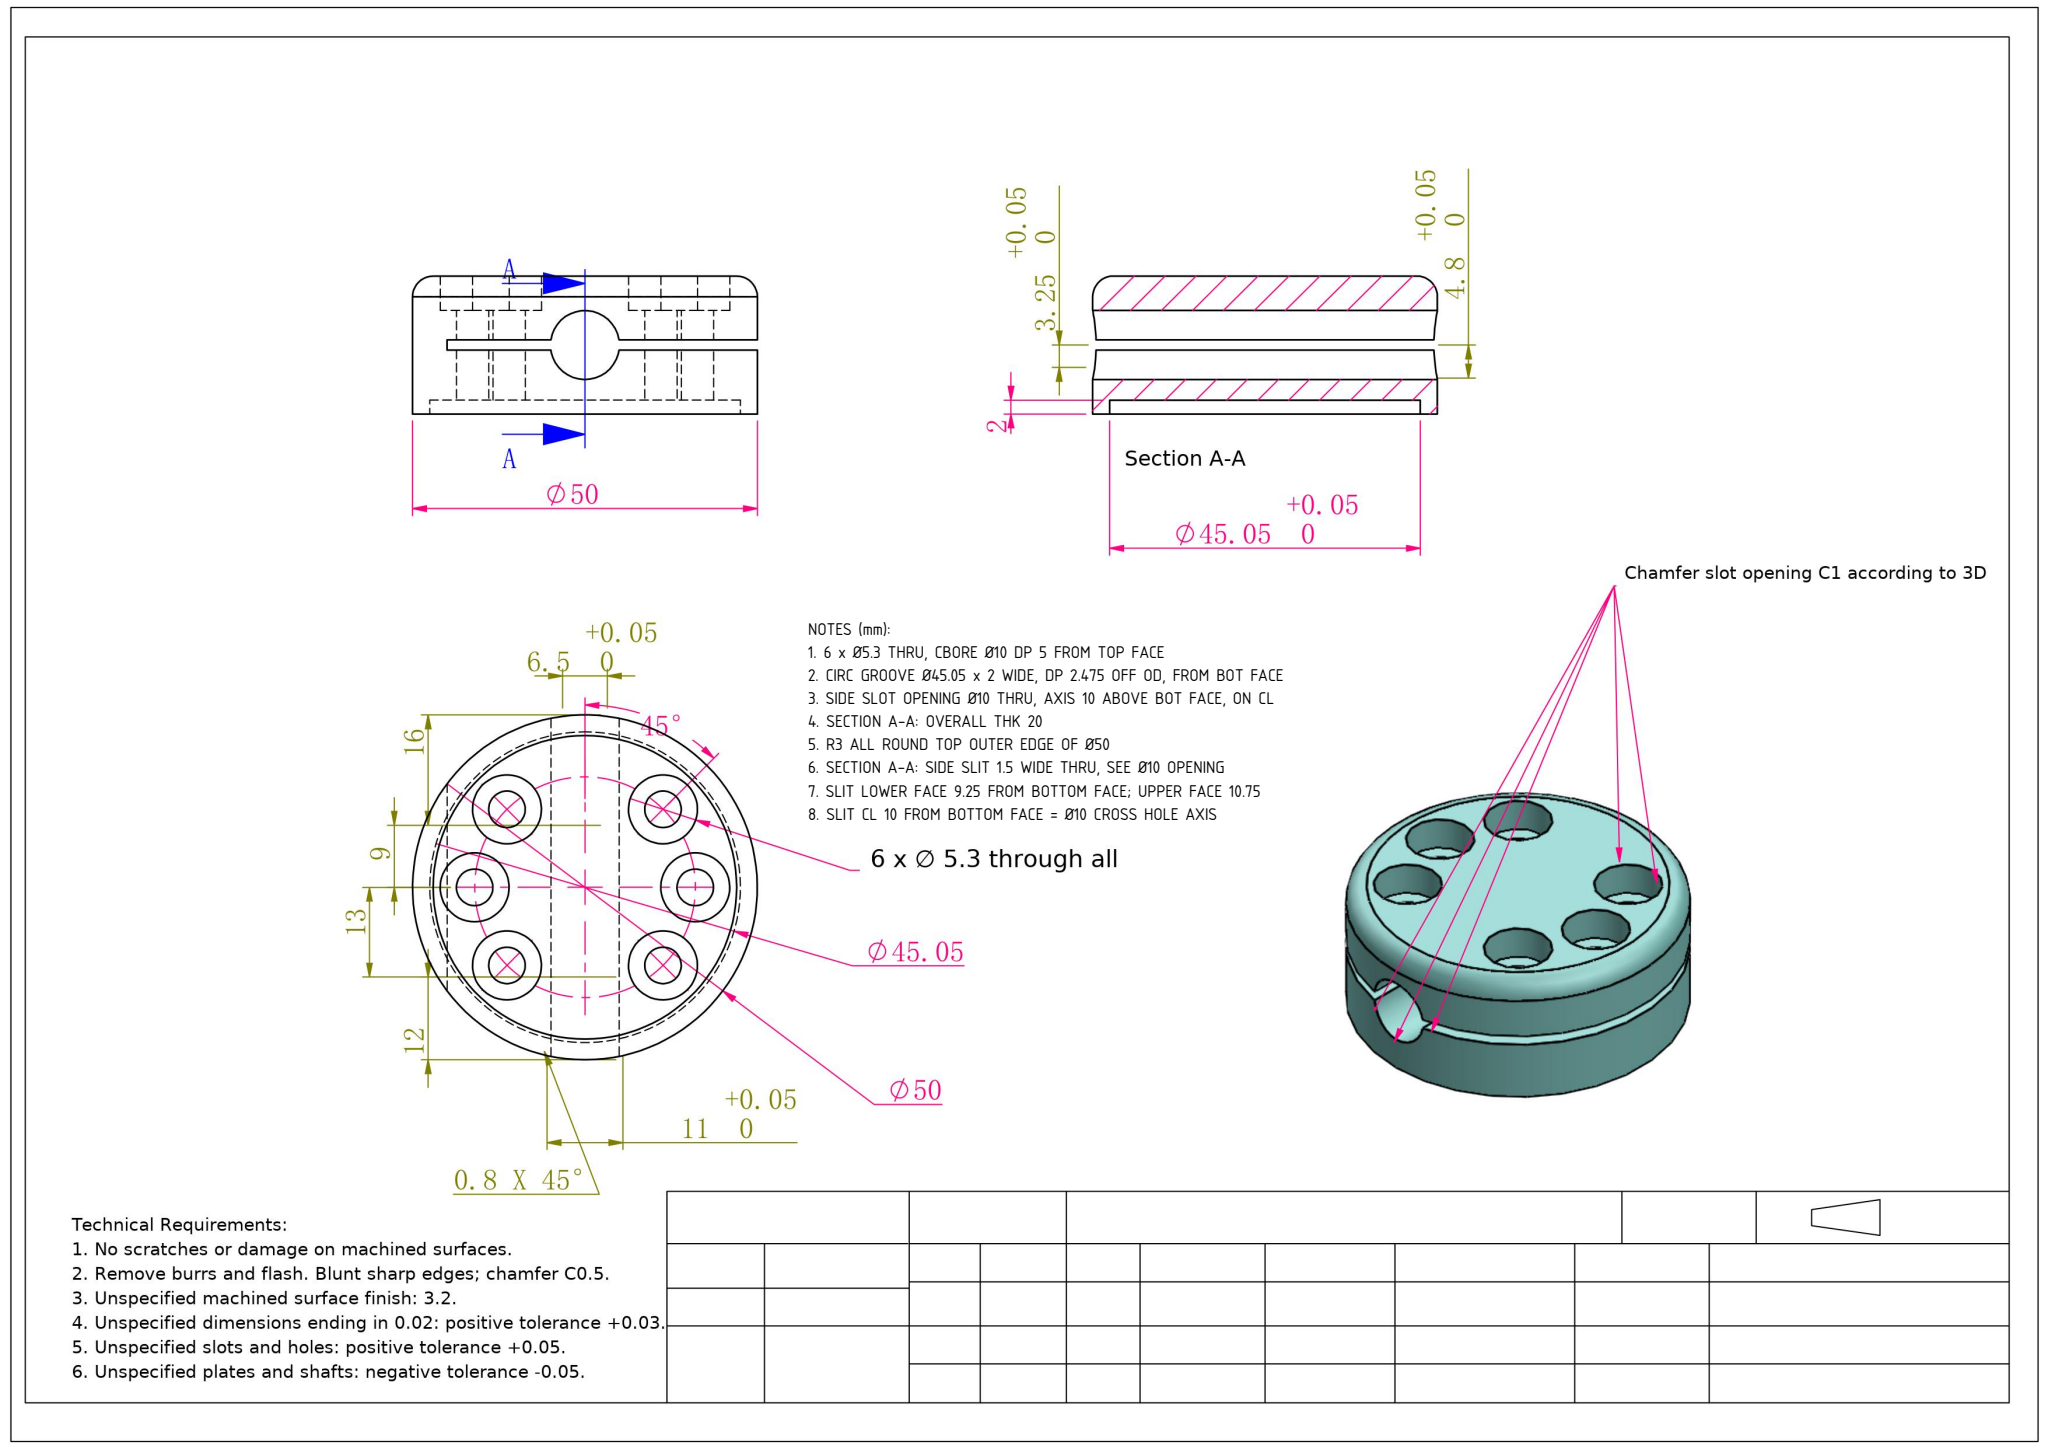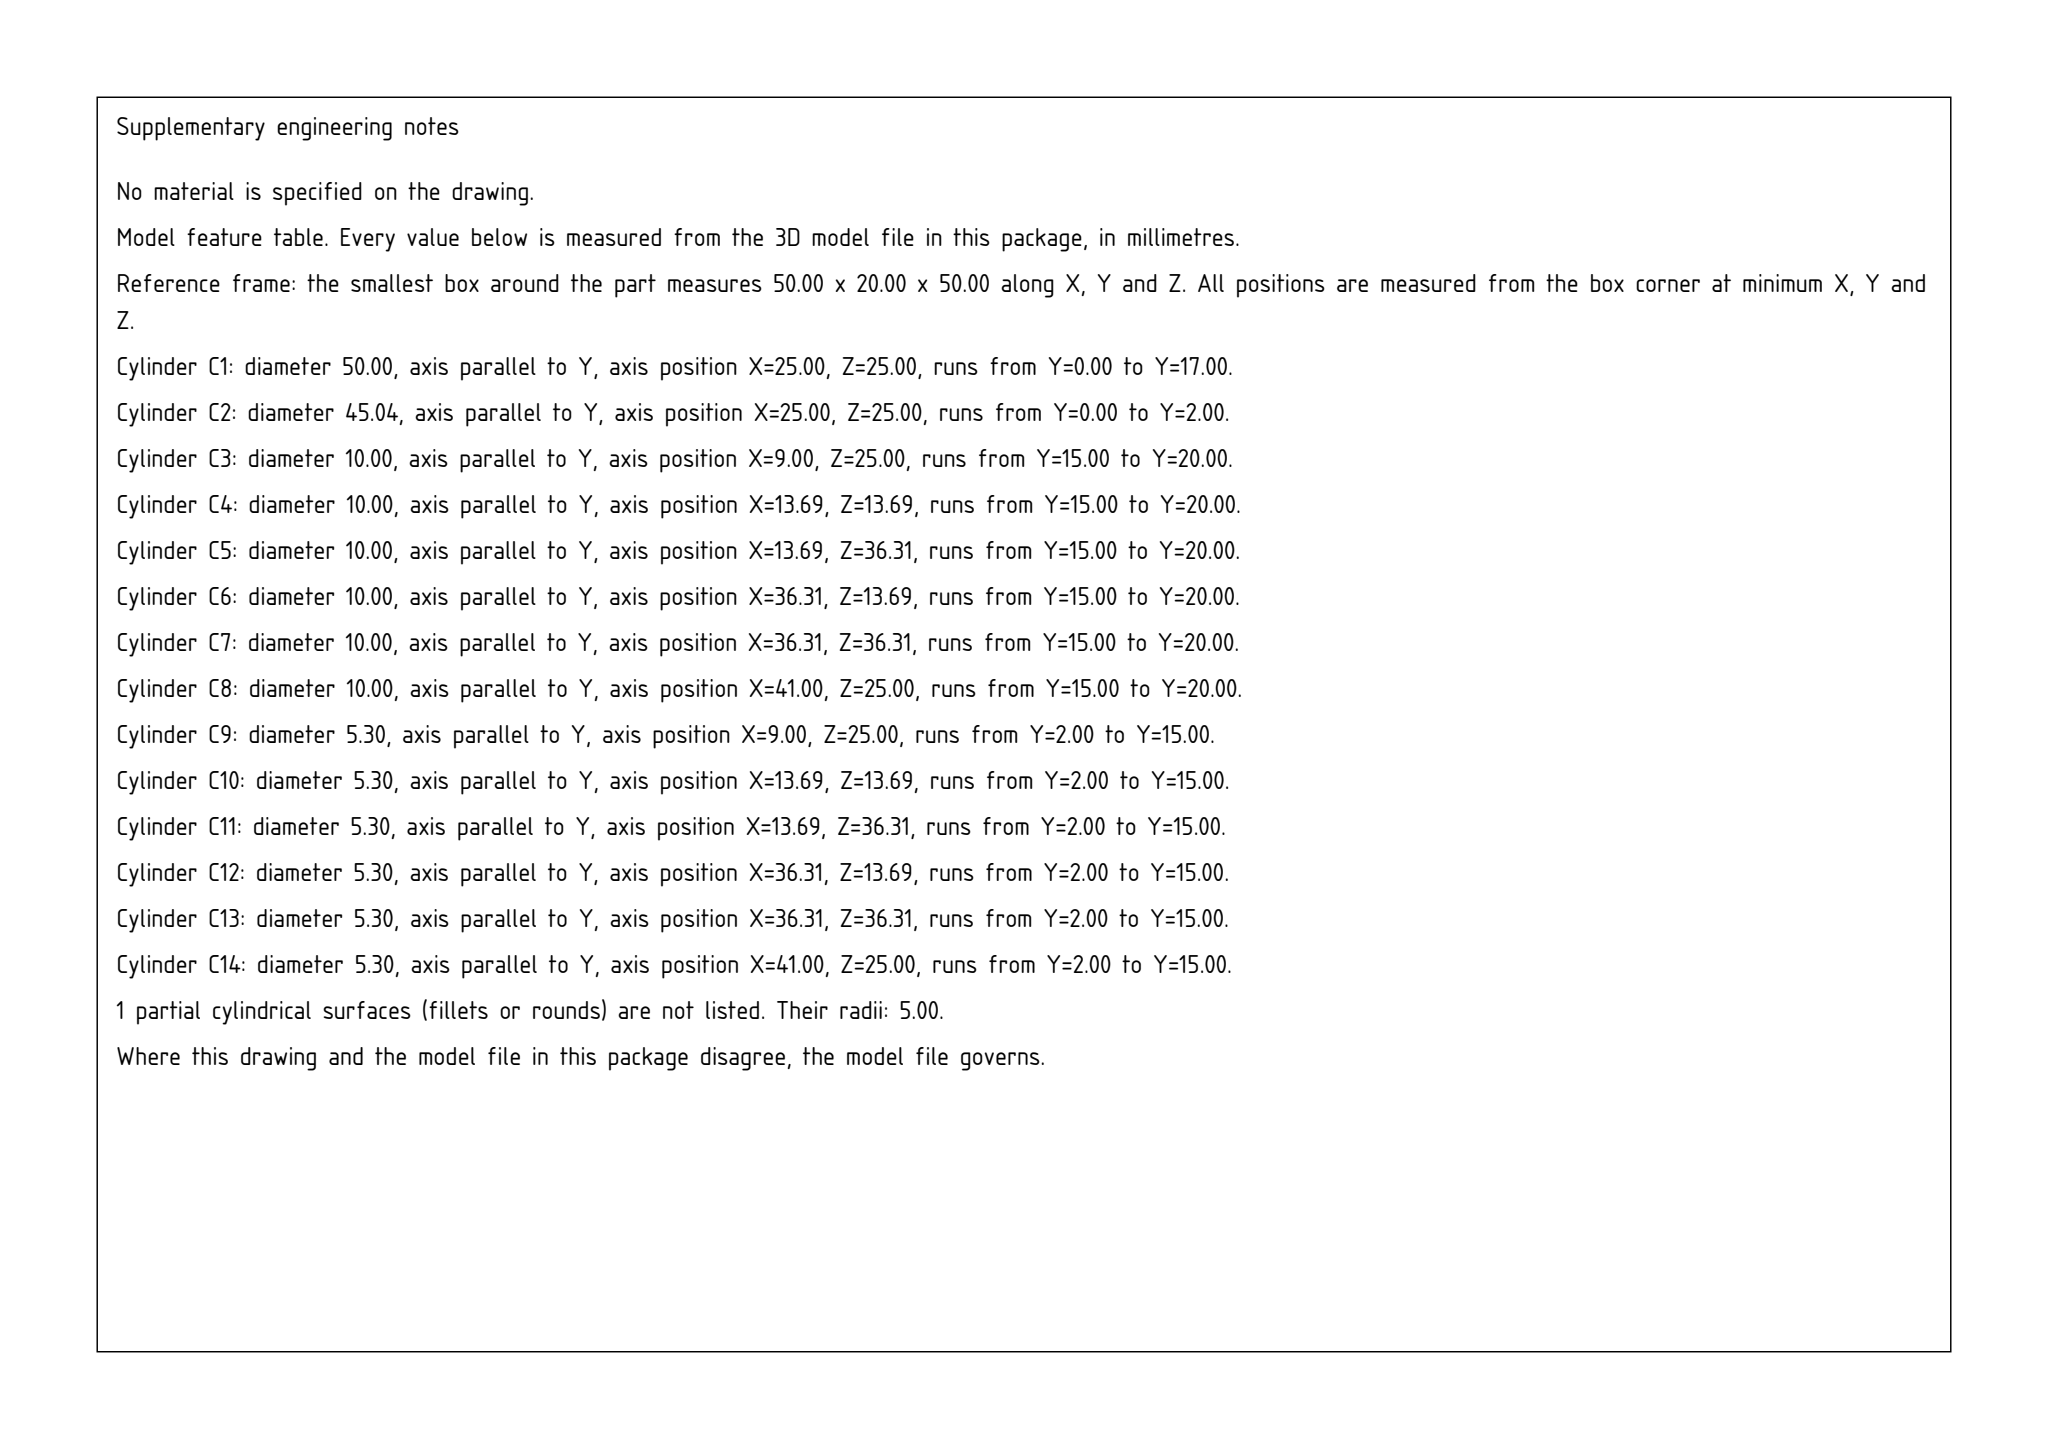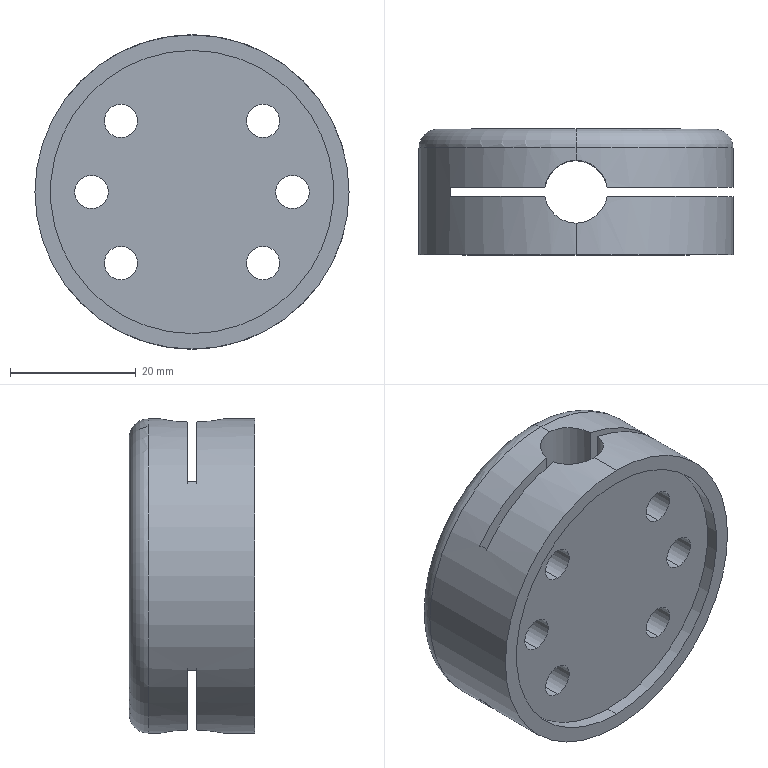Part | SolidWorks | mm | 1 solid | 59 faces | box 50 x 20 x 50 mm | volume 25951 mm3 | cylinder 43 | plane 14 | torus 2 | commonest cylinder face diameters 5.3 x24 10 x14 50 x3 45.05 x2
Drawing notes:
6 x Ø5.3 THRU, CBORE Ø10 DP 5 FROM TOP FACE | from the solid: Ø5.3 y-axis holes thru plate; Ø10 y-axis cyls len 5.0 from top y=20 to cbore floors at y=15 (6x)
CIRC GROOVE Ø45.05 x 2 WIDE, DP 2.475 OFF OD, FROM BOT FACE | from the solid: Ø45.05 y-axis cyl len 2.0 between y-planes 0 and 2; depth=(50-45.05)/2=2.475 off Ø50 OD
SIDE SLOT OPENING Ø10 THRU, AXIS 10 ABOVE BOT FACE, ON CL | from the solid: Ø10 z-axis cyl len 50 thru part, center x=27.06 (part CL), y=10.0 from bottom face y=0
SECTION A-A: OVERALL THK 20 | from the solid: bbox_xyz y-extent = 20.0 (planes y=0 to y=20)
R3 ALL ROUND TOP OUTER EDGE OF Ø50 | from the solid: fillet_radii [3.0,2]; Ø50 cyl ends y=17, top face y=20 (17+3=20)
SECTION A-A: SIDE SLIT 1.5 WIDE THRU, SEE Ø10 OPENING | from the solid: y-planes at 9.25 and 10.75 bound the gap: 10.75-9.25 = 1.5 wide slit
SLIT LOWER FACE 9.25 FROM BOTTOM FACE; UPPER FACE 10.75 | from the solid: axis_planes y=9.25 (2) and y=10.75 (2), datum y=0 bottom face
SLIT CL 10 FROM BOTTOM FACE = Ø10 CROSS HOLE AXIS | from the solid: Ø10 cyl axis y=10.0, midway between y=9.25 and y=10.75